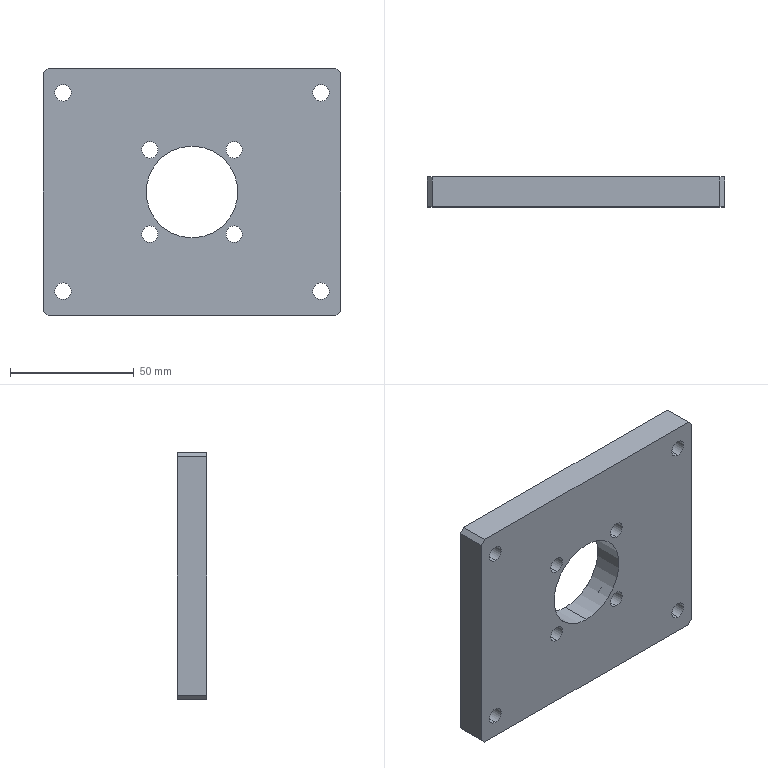Component | SolidWorks | 140507-L01M08U05-2-P01-1 | 1 solid | 52 faces | box 120 x 12 x 100 mm | volume 124603 mm3 | cylinder 34 | plane 18 | commonest cylinder face diameters 11 x16 6.6 x16 37 x2
build123d program:
from build123d import *

# Parameters (mm, degrees)
SKETCH1_W                                       = 120
SKETCH1_H                                       = 100
BOSS_EXTRUDE1_DEPTH                             = 12
CHAMFER1_SIZE                                   = 2
M6_HEX_SOCKET_HEAD_CAP_SCREW_CBORE1_D           = 6.6
M6_HEX_SOCKET_HEAD_CAP_SCREW_CBORE1_CBORE_D     = 11
M6_HEX_SOCKET_HEAD_CAP_SCREW_CBORE1_CBORE_DEPTH = 6.4
SKETCH4_R                                       = 18.5
CUT_EXTRUDE1_DEPTH                              = 12
M6_HEX_SOCKET_HEAD_CAP_SCREW_CBORE2_D           = 6.6
M6_HEX_SOCKET_HEAD_CAP_SCREW_CBORE2_CBORE_D     = 11
M6_HEX_SOCKET_HEAD_CAP_SCREW_CBORE2_CBORE_DEPTH = 6.4


with BuildPart() as part:
    # Sketch1 → Boss-Extrude1 (new body)
    with BuildSketch(Plane(origin=(0, 0, 0), x_dir=(1, 0, 0), z_dir=(0, 1, 0))):
        Rectangle(SKETCH1_W, SKETCH1_H)
    extrude(amount=BOSS_EXTRUDE1_DEPTH)

    # Chamfer1
    chamfer1_edges = [part.edges().sort_by_distance(p)[0] for p in [
        (60, 6, 50),
        (-60, 6, 50),
        (-60, 6, -50),
        (60, 6, -50),
    ]]
    chamfer(chamfer1_edges, length=CHAMFER1_SIZE)

    # M6 Hex Socket Head Cap Screw CBORE1 (through all)
    with Locations(Plane(origin=(0, 12, 0), x_dir=(1, 0, 0), z_dir=(0, 1, 0))):
        with Locations((-52, 40), (-52, -40), (52, -40), (52, 40)):
            CounterBoreHole(M6_HEX_SOCKET_HEAD_CAP_SCREW_CBORE1_D / 2, M6_HEX_SOCKET_HEAD_CAP_SCREW_CBORE1_CBORE_D / 2, M6_HEX_SOCKET_HEAD_CAP_SCREW_CBORE1_CBORE_DEPTH)

    # Sketch4 → Cut-Extrude1 (cut)
    with BuildSketch(Plane(origin=(0, 12, 0), x_dir=(1, 0, 0), z_dir=(0, 1, 0))):
        with Locations(Location((0, 0, 0), (0, 0, 270))):
            Circle(SKETCH4_R)
    extrude(amount=-CUT_EXTRUDE1_DEPTH, mode=Mode.SUBTRACT)

    # M6 Hex Socket Head Cap Screw CBORE2 (through all)
    with Locations(Plane(origin=(0, 12, 0), x_dir=(1, 0, 0), z_dir=(0, 1, 0))):
        with Locations((-17, 17), (-17, -17), (17, -17), (17, 17)):
            CounterBoreHole(M6_HEX_SOCKET_HEAD_CAP_SCREW_CBORE2_D / 2, M6_HEX_SOCKET_HEAD_CAP_SCREW_CBORE2_CBORE_D / 2, M6_HEX_SOCKET_HEAD_CAP_SCREW_CBORE2_CBORE_DEPTH)


solid = part.part

# Placed as in the assembly
solid = solid.moved(Location((17.055, -1.656, -21.398), (0, 0, 0)))